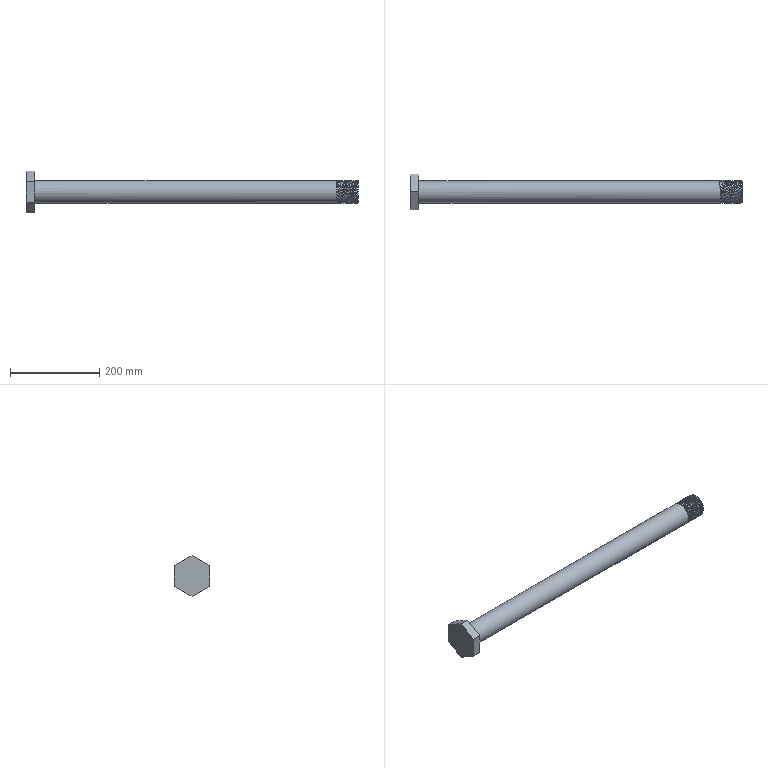Component | NX | PIN_SHAFT_2_5 | 1 solid | 23 faces | volume 1531080 mm3 | cylinder 11 | plane 10 | spline 2 | commonest cylinder face diameters 50 x10 48.5 x1